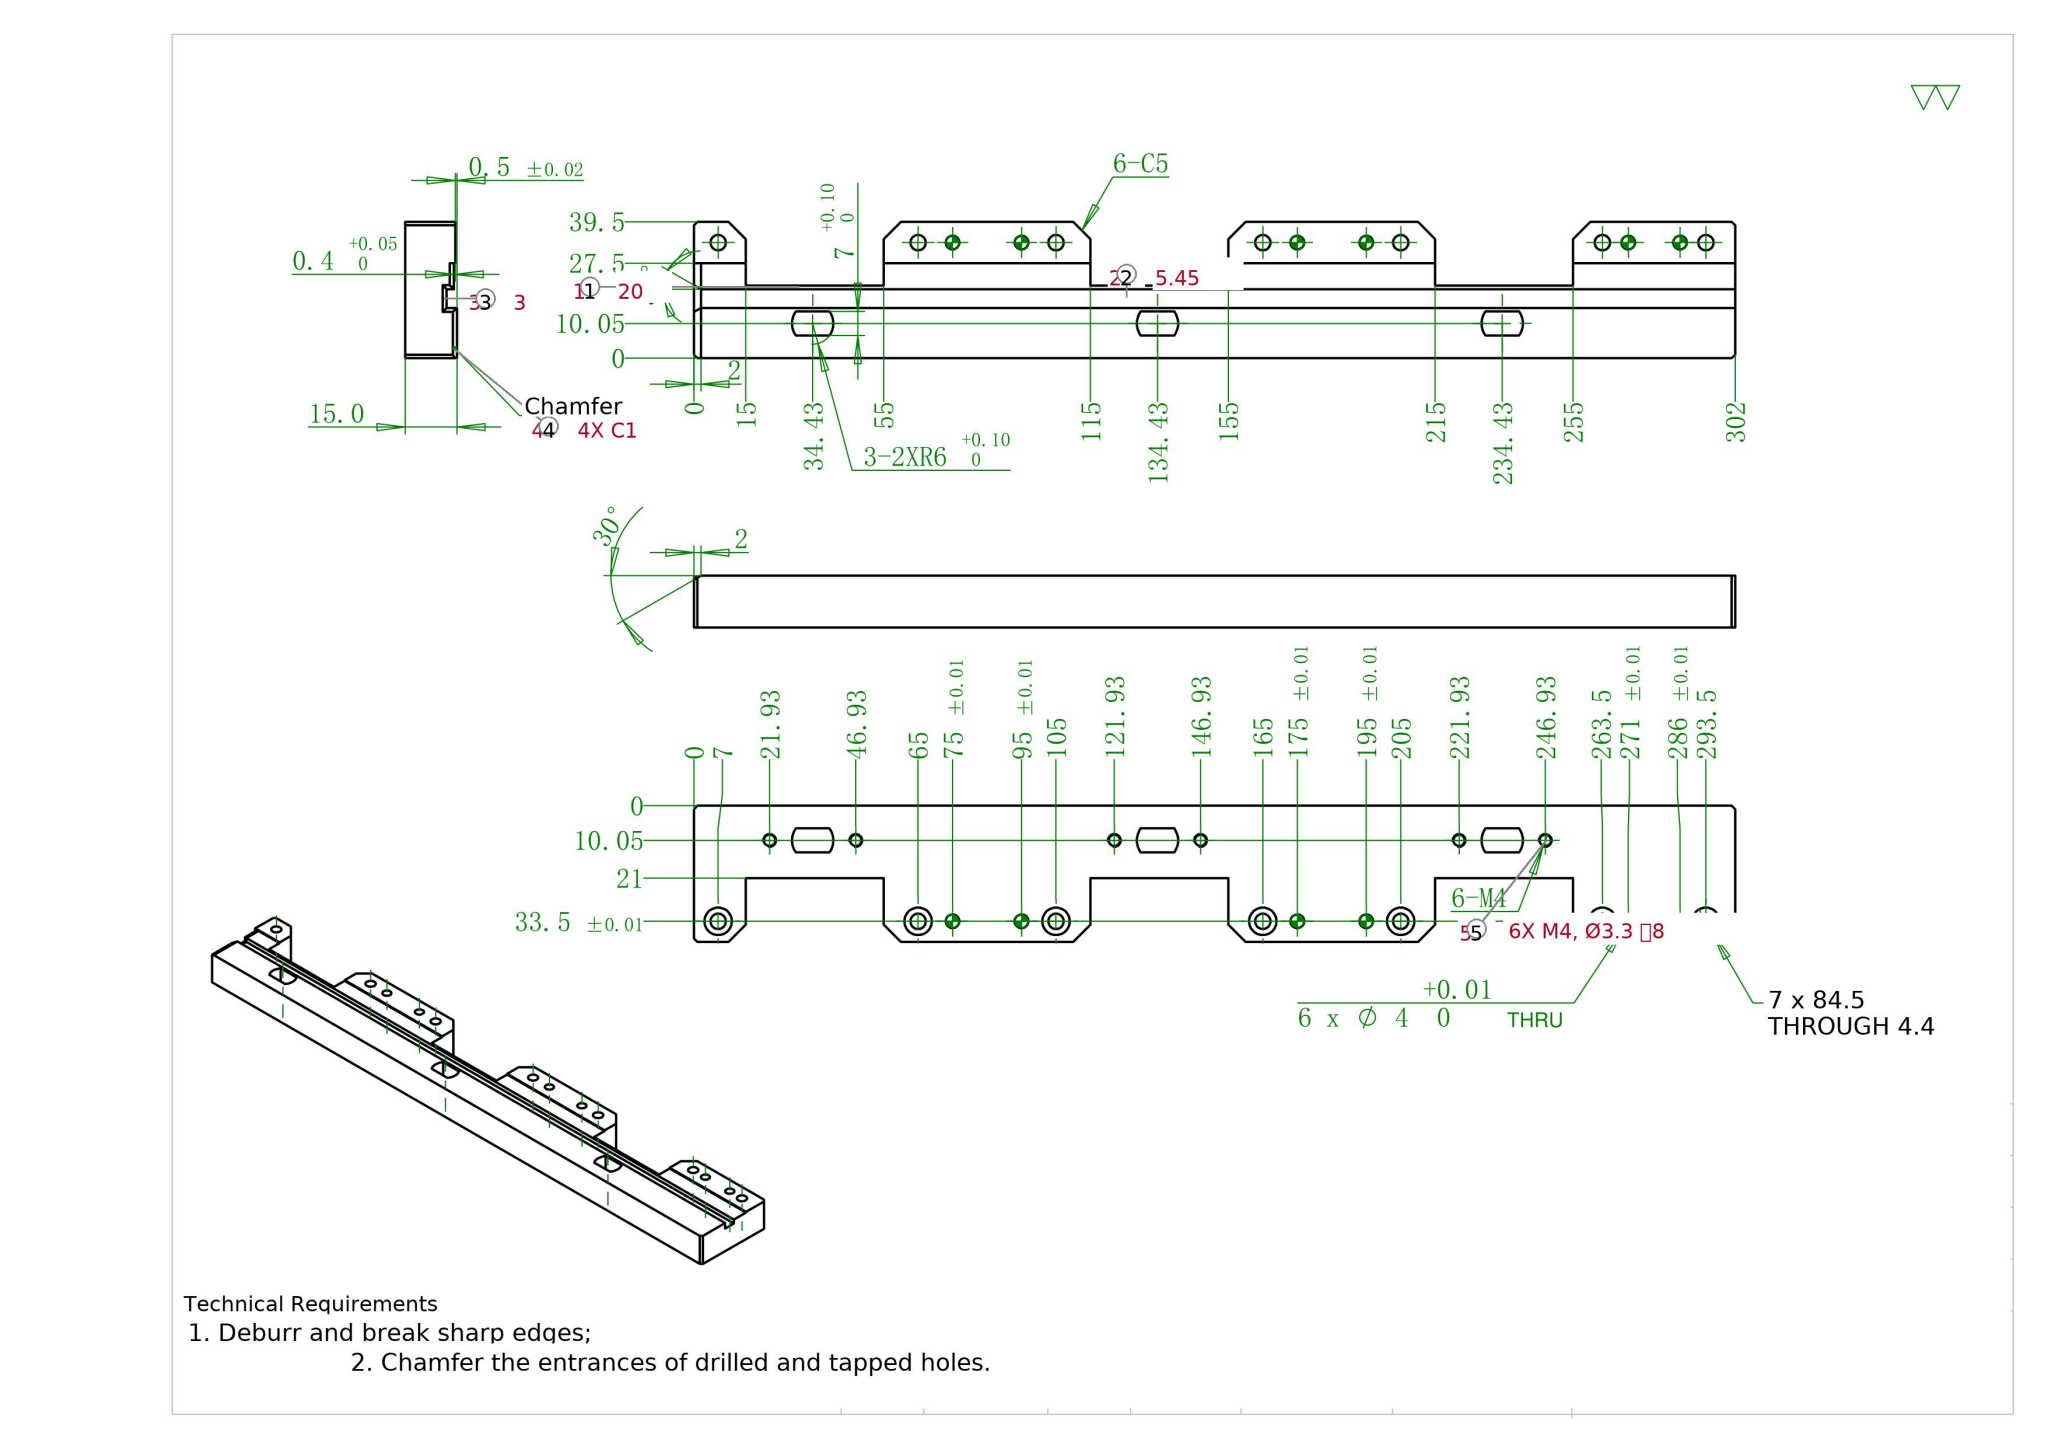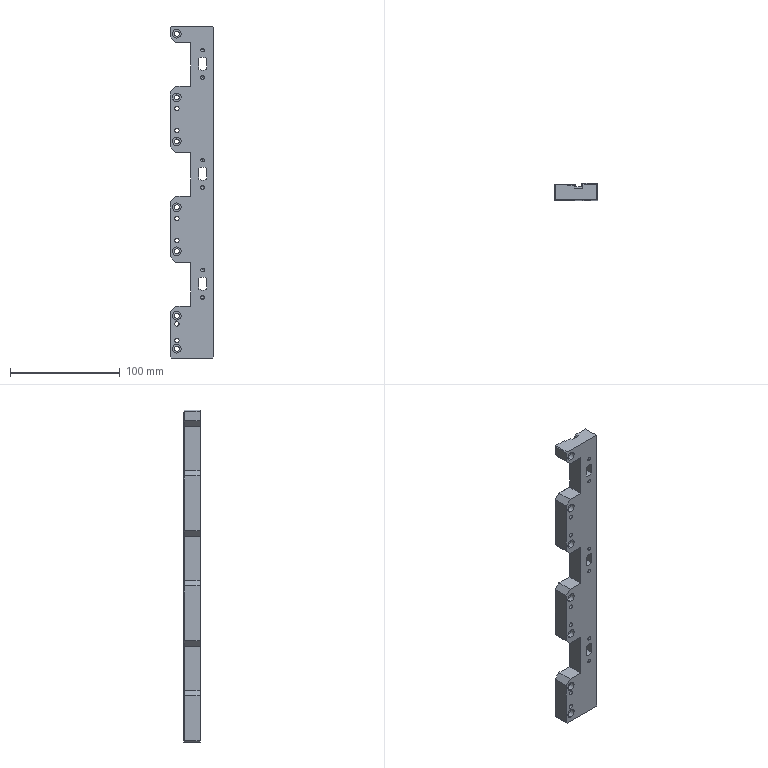Part | SolidWorks | mm | 1 solid | 128 faces | box 39.5 x 15 x 302 mm | volume 129368 mm3 | cylinder 58 | plane 58 | cone 12 | commonest cylinder face diameters 8 x14 4.5 x14 3.3 x12 4 x12 12 x6
build123d program:
from build123d import *
from OCP.BRepFilletAPI import BRepFilletAPI_MakeChamfer

# Parameters (mm, degrees)
BOSS_EXTRUDE1_DEPTH                             = 202
SKETCH2_W                                       = 19.5
SKETCH2_H                                       = 202
CUT_EXTRUDE1_DEPTH                              = 0.5
BOSS_EXTRUDE2_DEPTH                             = 100
CUT_EXTRUDE2_DEPTH                              = 207.372
LPATTERN1_COUNT                                 = 3
LPATTERN1_PITCH                                 = 100
SKETCH4_W                                       = 18.5
SKETCH4_H                                       = 40
CUT_EXTRUDE3_DEPTH                              = 207.372
LPATTERN2_COUNT                                 = 3
LPATTERN2_PITCH                                 = 100
M4_HEX_SOCKET_HEAD_CAP_SCREW_CBORE1_D           = 4.5
M4_HEX_SOCKET_HEAD_CAP_SCREW_CBORE1_CBORE_D     = 8
M4_HEX_SOCKET_HEAD_CAP_SCREW_CBORE1_CBORE_DEPTH = 4.4
F_4_0_4_DIAMETER_HOLE1_D                        = 4
CHAMFER1_SIZE                                   = 5
M4_TAPPED_HOLE1_D                               = 3.3
M4_TAPPED_HOLE1_DEPTH                           = 8
M4_TAPPED_HOLE1_TIP                             = 0.9914
SKETCH12_W                                      = 7.5
SKETCH12_H                                      = 0.4
CUT_EXTRUDE4_DEPTH                              = 305.941
CHAMFER2_SIZE                                   = 1
CHAMFER3_SIZE                                   = 2
CHAMFER3_SIZE2                                  = 1.155


with BuildPart() as part:
    # Sketch1 → Boss-Extrude1 (new body)
    with BuildSketch(Plane.XY):
        Polygon((0, 0), (0, 15), (19.5, 15), (19.5, 12), (24.95, 12), (24.95, 15), (39.5, 15), (39.5, 0), align=None)
    extrude(amount=BOSS_EXTRUDE1_DEPTH)

    # Sketch2 → Cut-Extrude1 (cut)
    with BuildSketch(Plane(origin=(0, 15, 0), x_dir=(1, 0, 0), z_dir=(0, 1, 0))):
        with Locations((9.75, -101)):
            Rectangle(SKETCH2_W, SKETCH2_H)
    extrude(amount=-CUT_EXTRUDE1_DEPTH, mode=Mode.SUBTRACT)

    # Sketch11 → Boss-Extrude2 (add)
    with BuildSketch(Plane(origin=(0, 0, 0), x_dir=(-1, 0, 0), z_dir=(0, 0, -1))):
        Polygon((0, 0), (0, 14.5), (-19.5, 14.5), (-19.5, 12), (-24.95, 12), (-24.95, 15), (-39.5, 15), (-39.5, 0), align=None)
    extrude(amount=BOSS_EXTRUDE2_DEPTH)

    # Sketch3 → Cut-Extrude2 (cut, through all)
    with BuildSketch(Plane.XZ):
        with BuildLine():
            Line((32.95, 172.443), (32.95, 162.697))
            ThreePointArc((32.95, 162.697), (29.45, 161.57), (25.95, 162.697))
            Line((25.95, 162.697), (25.95, 172.443))
            ThreePointArc((25.95, 172.443), (29.45, 173.57), (32.95, 172.443))
        make_face()
    cut_extrude2 = extrude(amount=-CUT_EXTRUDE2_DEPTH, mode=Mode.SUBTRACT)

    # LPattern1: Cut-Extrude2 ×3
    with Locations(*[(0, 0, -i * LPATTERN1_PITCH) for i in range(1, LPATTERN1_COUNT)]):
        add(cut_extrude2, mode=Mode.SUBTRACT)

    # Sketch4 → Cut-Extrude3 (cut, through all)
    with BuildSketch(Plane.XZ):
        with Locations((9.25, 167)):
            Rectangle(SKETCH4_W, SKETCH4_H)
    cut_extrude3 = extrude(amount=-CUT_EXTRUDE3_DEPTH, mode=Mode.SUBTRACT)

    # LPattern2: Cut-Extrude3 ×3
    with Locations(*[(0, 0, -i * LPATTERN2_PITCH) for i in range(1, LPATTERN2_COUNT)]):
        add(cut_extrude3, mode=Mode.SUBTRACT)

    # M4 Hex Socket Head Cap Screw CBORE1 (through all)
    with Locations(Plane(origin=(0, 0, 0), x_dir=(-1, 0, 0), z_dir=(0, -1, 0))):
        with Locations((-6, 3), (-6, -37), (-6, -97), (-6, -195), (-6, -137), (-6, 61.5), (-6, 91.5)):
            CounterBoreHole(M4_HEX_SOCKET_HEAD_CAP_SCREW_CBORE1_D / 2, M4_HEX_SOCKET_HEAD_CAP_SCREW_CBORE1_CBORE_D / 2, M4_HEX_SOCKET_HEAD_CAP_SCREW_CBORE1_CBORE_DEPTH)

    # 4.0 _4_ Diameter Hole1 (through all)
    with Locations(Plane(origin=(0, 0, 0), x_dir=(-1, 0, 0), z_dir=(0, -1, 0))):
        with Locations((-6, -127), (-6, -107), (-6, -27), (-6, -7), (-6, 69), (-6, 84)):
            Hole(F_4_0_4_DIAMETER_HOLE1_D / 2)

    # Chamfer1
    chamfer1_edges = [part.edges().sort_by_distance(p)[0] for p in [
        (0, 7.25, 147),
        (0, 7.25, 187),
        (0, 7.25, 47),
        (0, 7.25, 87),
        (0, 7.25, -53),
        (0, 7.25, -13),
    ]]
    chamfer(chamfer1_edges, length=CHAMFER1_SIZE)

    # M4 Tapped Hole1
    with Locations(Plane(origin=(0, 0, 0), x_dir=(-1, 0, 0), z_dir=(0, -1, 0))):
        with Locations((-29.45, -180.07), (-29.45, -155.07), (-29.45, -80.07), (-29.45, -55.07), (-29.45, 19.93), (-29.45, 44.93)):
            Hole(M4_TAPPED_HOLE1_D / 2, depth=M4_TAPPED_HOLE1_DEPTH)
            with Locations((0, 0, -(M4_TAPPED_HOLE1_DEPTH + M4_TAPPED_HOLE1_TIP / 2))):  # 118° drill point
                Cone(0, M4_TAPPED_HOLE1_D / 2, M4_TAPPED_HOLE1_TIP, mode=Mode.SUBTRACT)

    # Sketch12 → Cut-Extrude4 (cut, through all)
    with BuildSketch(Plane(origin=(0, 0, -100), x_dir=(-1, 0, 0), z_dir=(0, 0, -1))):
        with Locations((-15.75, 14.3)):
            Rectangle(SKETCH12_W, SKETCH12_H)
    extrude(amount=-CUT_EXTRUDE4_DEPTH, mode=Mode.SUBTRACT)

    # Chamfer2
    chamfer2_edges = [part.edges().sort_by_distance(p)[0] for p in [
        (0, 7.25, 202),
        (0, 7.25, -100),
        (39.5, 7.5, -100),
        (39.5, 7.5, 202),
    ]]
    chamfer(chamfer2_edges, length=CHAMFER2_SIZE)

    # Chamfer3: one chamfer whose edges measure the first distance from different faces: ONE call of the kernel's chamfer builder (chamfer() names one face for all edges)
    chamfer3_edges_1 = [part.edges().sort_by_distance(p)[0] for p in [
        (31.725, 15, 202),
    ]]
    chamfer3_side_1 = [part.faces().sort_by_distance(p)[0] for p in [
        (32.381, 15, 50.056),
    ]]
    chamfer3_edges_2 = [part.edges().sort_by_distance(p)[0] for p in [
        (24.95, 13.5, 202),
    ]]
    chamfer3_side_2 = [part.faces().sort_by_distance(p)[0] for p in [
        (24.95, 13.5, 51),
    ]]
    chamfer3_edges_3 = [part.edges().sort_by_distance(p)[0] for p in [
        (22.225, 12, 202),
    ]]
    chamfer3_side_3 = [part.faces().sort_by_distance(p)[0] for p in [
        (22.225, 12, 51),
    ]]
    chamfer3_edges_4 = [part.edges().sort_by_distance(p)[0] for p in [
        (19.5, 13.05, 202),
    ]]
    chamfer3_side_4 = [part.faces().sort_by_distance(p)[0] for p in [
        (19.5, 13.05, 51),
    ]]
    chamfer3_edges_5 = [part.edges().sort_by_distance(p)[0] for p in [
        (15.75, 14.1, 202),
    ]]
    chamfer3_side_5 = [part.faces().sort_by_distance(p)[0] for p in [
        (16.013, 14.1, 42.596),
    ]]
    chamfer3 = BRepFilletAPI_MakeChamfer(part.part.solid().wrapped)
    for e in chamfer3_edges_1:
        chamfer3.Add(CHAMFER3_SIZE, CHAMFER3_SIZE2, e.wrapped, chamfer3_side_1[0].wrapped)  # the first distance lies on this face
    for e in chamfer3_edges_2:
        chamfer3.Add(CHAMFER3_SIZE, CHAMFER3_SIZE2, e.wrapped, chamfer3_side_2[0].wrapped)  # the first distance lies on this face
    for e in chamfer3_edges_3:
        chamfer3.Add(CHAMFER3_SIZE, CHAMFER3_SIZE2, e.wrapped, chamfer3_side_3[0].wrapped)  # the first distance lies on this face
    for e in chamfer3_edges_4:
        chamfer3.Add(CHAMFER3_SIZE, CHAMFER3_SIZE2, e.wrapped, chamfer3_side_4[0].wrapped)  # the first distance lies on this face
    for e in chamfer3_edges_5:
        chamfer3.Add(CHAMFER3_SIZE, CHAMFER3_SIZE2, e.wrapped, chamfer3_side_5[0].wrapped)  # the first distance lies on this face
    add(Compound.cast(chamfer3.Shape()), mode=Mode.REPLACE)


solid = part.part